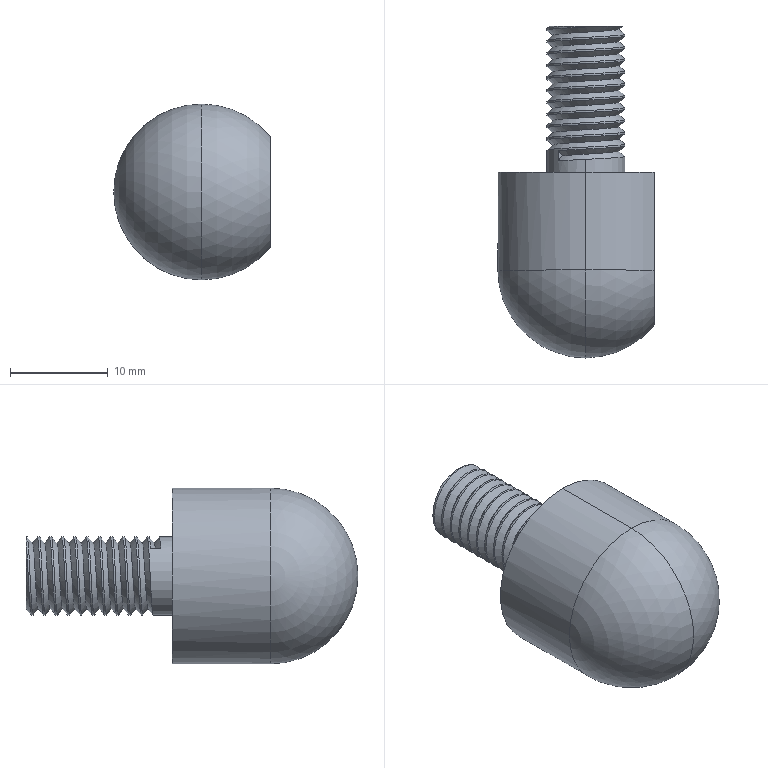Component | SolidWorks | HingeAssembly-1_Hinge1-2 | 1 solid | 38 faces | volume 4132 mm3 | cylinder 28 | plane 6 | sphere 2 | spline 2 | commonest cylinder face diameters 8 x25 18 x3